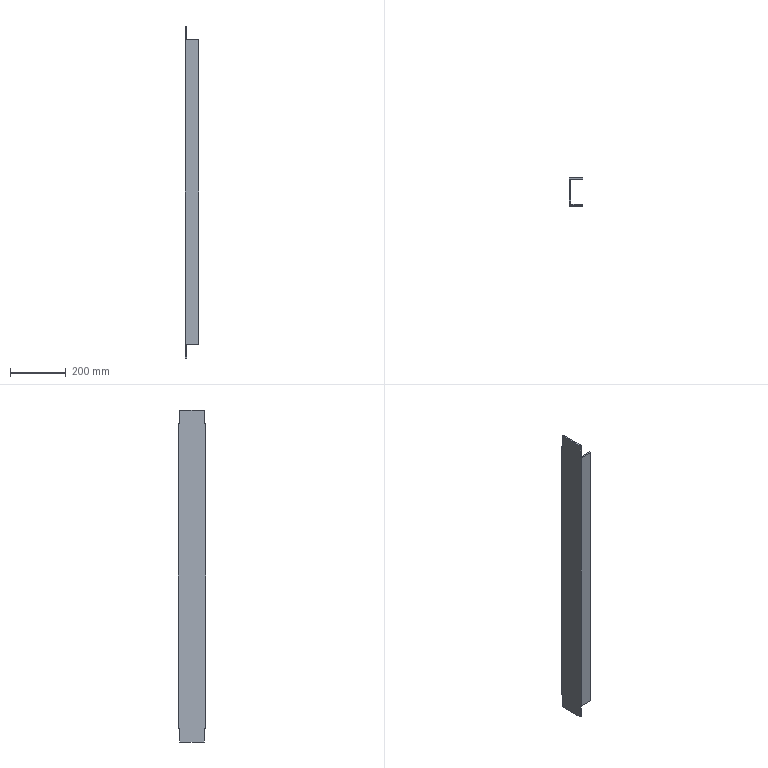Component | SolidWorks | 03LeftSideBase-2 | 1 solid | 28 faces | box 48 x 100 x 1189 mm | volume 1154848 mm3 | plane 18 | cylinder 10 | commonest cylinder face diameters 10 x10
build123d program:
from build123d import *

# Parameters (mm, degrees)
EXTRUDE_THIN1_DEPTH            = 1189
SKETCH2_W                      = 48
SKETCH2_H                      = 50
CUT_EXTRUDE1_DEPTH             = 5.5
SKETCH3_W                      = 48
SKETCH3_H                      = 50
CUT_EXTRUDE2_DEPTH             = 5.5
F_10_0_10_DIAMETER_HOLE1_D     = 10
F_10_0_10_DIAMETER_HOLE1_DEPTH = 5.5


with BuildPart() as part:
    # Sketch1 → Extrude-Thin1 (new body)
    with BuildSketch(Plane.XY):
        Polygon((48, 0), (0, 0), (0, 100), (48, 100), (48, 94.5), (5.5, 94.5), (5.5, 5.5), (48, 5.5), align=None)
    extrude(amount=EXTRUDE_THIN1_DEPTH)

    # Sketch2 → Cut-Extrude1 (cut)
    with BuildSketch(Plane(origin=(0, 100, 0), x_dir=(1, 0, 0), z_dir=(0, 1, 0))):
        with Locations((24, -1164)):
            Rectangle(SKETCH2_W, SKETCH2_H)
        with Locations((24, -25)):
            Rectangle(SKETCH2_W, SKETCH2_H)
    extrude(amount=-CUT_EXTRUDE1_DEPTH, mode=Mode.SUBTRACT)

    # Sketch3 → Cut-Extrude2 (cut)
    with BuildSketch(Plane.XZ):
        with Locations((24, 25)):
            Rectangle(SKETCH3_W, SKETCH3_H)
        with Locations((24, 1164)):
            Rectangle(SKETCH3_W, SKETCH3_H)
    extrude(amount=-CUT_EXTRUDE2_DEPTH, mode=Mode.SUBTRACT)

    # 10.0 _10_ Diameter Hole1
    with Locations(Plane(origin=(0, 100, 0), x_dir=(-1, 0, 0), z_dir=(0, 1, 0))):
        with Locations((-18, 194.5), (-18, 594.5), (-18, 994.5), (-18, 1126.5), (-18, 62.5)):
            Hole(F_10_0_10_DIAMETER_HOLE1_D / 2, depth=F_10_0_10_DIAMETER_HOLE1_DEPTH)


solid = part.part

# Placed as in the assembly
solid = solid.moved(Location((-123.527, -139.54, 42.607), (0, 0, 0)))
STEP:
#1=CARTESIAN_POINT('',(-4.155,-1.773,9.138));
#2=VERTEX_POINT('',#1);
#3=CARTESIAN_POINT('',(-4.155,-1.773,9.532));
#4=VERTEX_POINT('',#3);
#5=CARTESIAN_POINT('',(-4.155,-1.773,9.335));
#6=DIRECTION('',(0.,1.,0.));
#7=DIRECTION('',(0.,0.,1.));
#8=AXIS2_PLACEMENT_3D('',#5,#6,#7);
#9=CIRCLE('',#8,0.1969);
#10=EDGE_CURVE('',#2,#4,#9,.T.);
#11=ORIENTED_EDGE('',*,*,#10,.F.);
#12=CARTESIAN_POINT('',(-4.155,-1.557,9.138));
#13=VERTEX_POINT('',#12);
#14=CARTESIAN_POINT('',(-4.155,-1.557,9.138));
#15=DIRECTION('',(0.,1.,0.));
#16=VECTOR('',#15,39.37);
#17=LINE('',#14,#16);
#18=EDGE_CURVE('',#2,#13,#17,.T.);
#19=ORIENTED_EDGE('',*,*,#18,.T.);
#20=CARTESIAN_POINT('',(-4.155,-1.557,9.532));
#21=VERTEX_POINT('',#20);
#22=CARTESIAN_POINT('',(-4.155,-1.557,9.335));
#23=DIRECTION('',(0.,1.,0.));
#24=DIRECTION('',(0.,0.,1.));
#25=AXIS2_PLACEMENT_3D('',#22,#23,#24);
#26=CIRCLE('',#25,0.1969);
#27=EDGE_CURVE('',#13,#21,#26,.T.);
#28=ORIENTED_EDGE('',*,*,#27,.T.);
#29=CARTESIAN_POINT('',(-4.155,-1.557,9.532));
#30=DIRECTION('',(0.,1.,0.));
#31=VECTOR('',#30,39.37);
#32=LINE('',#29,#31);
#33=EDGE_CURVE('',#4,#21,#32,.T.);
#34=ORIENTED_EDGE('',*,*,#33,.F.);
#35=EDGE_LOOP('',(#11,#19,#28,#34));
#36=FACE_OUTER_BOUND('',#35,.T.);
#37=CARTESIAN_POINT('',(-4.155,-1.557,9.335));
#38=DIRECTION('',(0.,1.,0.));
#39=DIRECTION('',(0.,0.,1.));
#40=AXIS2_PLACEMENT_3D('',#37,#38,#39);
#41=CYLINDRICAL_SURFACE('',#40,0.1969);
#42=ADVANCED_FACE('',(#36),#41,.F.);
#43=CARTESIAN_POINT('',(-4.155,-1.773,24.886));
#44=VERTEX_POINT('',#43);
#45=CARTESIAN_POINT('',(-4.155,-1.773,25.28));
#46=VERTEX_POINT('',#45);
#47=CARTESIAN_POINT('',(-4.155,-1.773,25.083));
#48=DIRECTION('',(0.,1.,0.));
#49=DIRECTION('',(0.,0.,1.));
#50=AXIS2_PLACEMENT_3D('',#47,#48,#49);
#51=CIRCLE('',#50,0.1969);
#52=EDGE_CURVE('',#44,#46,#51,.T.);
#53=ORIENTED_EDGE('',*,*,#52,.F.);
#54=CARTESIAN_POINT('',(-4.155,-1.557,24.886));
#55=VERTEX_POINT('',#54);
#56=CARTESIAN_POINT('',(-4.155,-1.557,24.886));
#57=DIRECTION('',(0.,1.,0.));
#58=VECTOR('',#57,39.37);
#59=LINE('',#56,#58);
#60=EDGE_CURVE('',#44,#55,#59,.T.);
#61=ORIENTED_EDGE('',*,*,#60,.T.);
#62=CARTESIAN_POINT('',(-4.155,-1.557,25.28));
#63=VERTEX_POINT('',#62);
#64=CARTESIAN_POINT('',(-4.155,-1.557,25.083));
#65=DIRECTION('',(0.,1.,0.));
#66=DIRECTION('',(0.,0.,1.));
#67=AXIS2_PLACEMENT_3D('',#64,#65,#66);
#68=CIRCLE('',#67,0.1969);
#69=EDGE_CURVE('',#55,#63,#68,.T.);
#70=ORIENTED_EDGE('',*,*,#69,.T.);
#71=CARTESIAN_POINT('',(-4.155,-1.557,25.28));
#72=DIRECTION('',(0.,1.,0.));
#73=VECTOR('',#72,39.37);
#74=LINE('',#71,#73);
#75=EDGE_CURVE('',#46,#63,#74,.T.);
#76=ORIENTED_EDGE('',*,*,#75,.F.);
#77=EDGE_LOOP('',(#53,#61,#70,#76));
#78=FACE_OUTER_BOUND('',#77,.T.);
#79=CARTESIAN_POINT('',(-4.155,-1.557,25.083));
#80=DIRECTION('',(0.,1.,0.));
#81=DIRECTION('',(0.,0.,1.));
#82=AXIS2_PLACEMENT_3D('',#79,#80,#81);
#83=CYLINDRICAL_SURFACE('',#82,0.1969);
#84=ADVANCED_FACE('',(#78),#83,.F.);
#85=CARTESIAN_POINT('',(-4.155,-1.773,40.634));
#86=VERTEX_POINT('',#85);
#87=CARTESIAN_POINT('',(-4.155,-1.773,41.028));
#88=VERTEX_POINT('',#87);
#89=CARTESIAN_POINT('',(-4.155,-1.773,40.831));
#90=DIRECTION('',(0.,1.,0.));
#91=DIRECTION('',(0.,0.,1.));
#92=AXIS2_PLACEMENT_3D('',#89,#90,#91);
#93=CIRCLE('',#92,0.1969);
#94=EDGE_CURVE('',#86,#88,#93,.T.);
#95=ORIENTED_EDGE('',*,*,#94,.F.);
#96=CARTESIAN_POINT('',(-4.155,-1.557,40.634));
#97=VERTEX_POINT('',#96);
#98=CARTESIAN_POINT('',(-4.155,-1.557,40.634));
#99=DIRECTION('',(0.,1.,0.));
#100=VECTOR('',#99,39.37);
#101=LINE('',#98,#100);
#102=EDGE_CURVE('',#86,#97,#101,.T.);
#103=ORIENTED_EDGE('',*,*,#102,.T.);
#104=CARTESIAN_POINT('',(-4.155,-1.557,41.028));
#105=VERTEX_POINT('',#104);
#106=CARTESIAN_POINT('',(-4.155,-1.557,40.831));
#107=DIRECTION('',(0.,1.,0.));
#108=DIRECTION('',(0.,0.,1.));
#109=AXIS2_PLACEMENT_3D('',#106,#107,#108);
#110=CIRCLE('',#109,0.1969);
#111=EDGE_CURVE('',#97,#105,#110,.T.);
#112=ORIENTED_EDGE('',*,*,#111,.T.);
#113=CARTESIAN_POINT('',(-4.155,-1.557,41.028));
#114=DIRECTION('',(0.,1.,0.));
#115=VECTOR('',#114,39.37);
#116=LINE('',#113,#115);
#117=EDGE_CURVE('',#88,#105,#116,.T.);
#118=ORIENTED_EDGE('',*,*,#117,.F.);
#119=EDGE_LOOP('',(#95,#103,#112,#118));
#120=FACE_OUTER_BOUND('',#119,.T.);
#121=CARTESIAN_POINT('',(-4.155,-1.557,40.831));
#122=DIRECTION('',(0.,1.,0.));
#123=DIRECTION('',(0.,0.,1.));
#124=AXIS2_PLACEMENT_3D('',#121,#122,#123);
#125=CYLINDRICAL_SURFACE('',#124,0.1969);
#126=ADVANCED_FACE('',(#120),#125,.F.);
#127=CARTESIAN_POINT('',(-4.155,-1.773,45.831));
#128=VERTEX_POINT('',#127);
#129=CARTESIAN_POINT('',(-4.155,-1.773,46.225));
#130=VERTEX_POINT('',#129);
#131=CARTESIAN_POINT('',(-4.155,-1.773,46.028));
#132=DIRECTION('',(0.,1.,0.));
#133=DIRECTION('',(0.,0.,1.));
#134=AXIS2_PLACEMENT_3D('',#131,#132,#133);
#135=CIRCLE('',#134,0.1969);
#136=EDGE_CURVE('',#128,#130,#135,.T.);
#137=ORIENTED_EDGE('',*,*,#136,.F.);
#138=CARTESIAN_POINT('',(-4.155,-1.557,45.831));
#139=VERTEX_POINT('',#138);
#140=CARTESIAN_POINT('',(-4.155,-1.557,45.831));
#141=DIRECTION('',(0.,1.,0.));
#142=VECTOR('',#141,39.37);
#143=LINE('',#140,#142);
#144=EDGE_CURVE('',#128,#139,#143,.T.);
#145=ORIENTED_EDGE('',*,*,#144,.T.);
#146=CARTESIAN_POINT('',(-4.155,-1.557,46.225));
#147=VERTEX_POINT('',#146);
#148=CARTESIAN_POINT('',(-4.155,-1.557,46.028));
#149=DIRECTION('',(0.,1.,0.));
#150=DIRECTION('',(0.,0.,1.));
#151=AXIS2_PLACEMENT_3D('',#148,#149,#150);
#152=CIRCLE('',#151,0.1969);
#153=EDGE_CURVE('',#139,#147,#152,.T.);
#154=ORIENTED_EDGE('',*,*,#153,.T.);
#155=CARTESIAN_POINT('',(-4.155,-1.557,46.225));
#156=DIRECTION('',(0.,1.,0.));
#157=VECTOR('',#156,39.37);
#158=LINE('',#155,#157);
#159=EDGE_CURVE('',#130,#147,#158,.T.);
#160=ORIENTED_EDGE('',*,*,#159,.F.);
#161=EDGE_LOOP('',(#137,#145,#154,#160));
#162=FACE_OUTER_BOUND('',#161,.T.);
#163=CARTESIAN_POINT('',(-4.155,-1.557,46.028));
#164=DIRECTION('',(0.,1.,0.));
#165=DIRECTION('',(0.,0.,1.));
#166=AXIS2_PLACEMENT_3D('',#163,#164,#165);
#167=CYLINDRICAL_SURFACE('',#166,0.1969);
#168=ADVANCED_FACE('',(#162),#167,.F.);
#169=CARTESIAN_POINT('',(-4.155,-1.773,3.941));
#170=VERTEX_POINT('',#169);
#171=CARTESIAN_POINT('',(-4.155,-1.773,4.335));
#172=VERTEX_POINT('',#171);
#173=CARTESIAN_POINT('',(-4.155,-1.773,4.138));
#174=DIRECTION('',(0.,1.,0.));
#175=DIRECTION('',(0.,0.,1.));
#176=AXIS2_PLACEMENT_3D('',#173,#174,#175);
#177=CIRCLE('',#176,0.1969);
#178=EDGE_CURVE('',#170,#172,#177,.T.);
#179=ORIENTED_EDGE('',*,*,#178,.F.);
#180=CARTESIAN_POINT('',(-4.155,-1.557,3.941));
#181=VERTEX_POINT('',#180);
#182=CARTESIAN_POINT('',(-4.155,-1.557,3.941));
#183=DIRECTION('',(0.,1.,0.));
#184=VECTOR('',#183,39.37);
#185=LINE('',#182,#184);
#186=EDGE_CURVE('',#170,#181,#185,.T.);
#187=ORIENTED_EDGE('',*,*,#186,.T.);
#188=CARTESIAN_POINT('',(-4.155,-1.557,4.335));
#189=VERTEX_POINT('',#188);
#190=CARTESIAN_POINT('',(-4.155,-1.557,4.138));
#191=DIRECTION('',(0.,1.,0.));
#192=DIRECTION('',(0.,0.,1.));
#193=AXIS2_PLACEMENT_3D('',#190,#191,#192);
#194=CIRCLE('',#193,0.1969);
#195=EDGE_CURVE('',#181,#189,#194,.T.);
#196=ORIENTED_EDGE('',*,*,#195,.T.);
#197=CARTESIAN_POINT('',(-4.155,-1.557,4.335));
#198=DIRECTION('',(0.,1.,0.));
#199=VECTOR('',#198,39.37);
#200=LINE('',#197,#199);
#201=EDGE_CURVE('',#172,#189,#200,.T.);
#202=ORIENTED_EDGE('',*,*,#201,.F.);
#203=EDGE_LOOP('',(#179,#187,#196,#202));
#204=FACE_OUTER_BOUND('',#203,.T.);
#205=CARTESIAN_POINT('',(-4.155,-1.557,4.138));
#206=DIRECTION('',(0.,1.,0.));
#207=DIRECTION('',(0.,0.,1.));
#208=AXIS2_PLACEMENT_3D('',#205,#206,#207);
#209=CYLINDRICAL_SURFACE('',#208,0.1969);
#210=ADVANCED_FACE('',(#204),#209,.F.);
#211=CARTESIAN_POINT('',(-4.863,-5.277,48.488));
#212=VERTEX_POINT('',#211);
#213=CARTESIAN_POINT('',(-4.647,-5.277,48.488));
#214=VERTEX_POINT('',#213);
#215=CARTESIAN_POINT('',(-2.974,-5.277,48.488));
#216=DIRECTION('',(1.,-0.,0.));
#217=VECTOR('',#216,39.37);
#218=LINE('',#215,#217);
#219=EDGE_CURVE('',#212,#214,#218,.T.);
#220=ORIENTED_EDGE('',*,*,#219,.T.);
#221=CARTESIAN_POINT('',(-4.647,-1.773,48.488));
#222=VERTEX_POINT('',#221);
#223=CARTESIAN_POINT('',(-4.647,-5.494,48.488));
#224=DIRECTION('',(0.,1.,0.));
#225=VECTOR('',#224,39.37);
#226=LINE('',#223,#225);
#227=EDGE_CURVE('',#214,#222,#226,.T.);
#228=ORIENTED_EDGE('',*,*,#227,.T.);
#229=CARTESIAN_POINT('',(-4.863,-1.773,48.488));
#230=VERTEX_POINT('',#229);
#231=CARTESIAN_POINT('',(-2.974,-1.773,48.488));
#232=DIRECTION('',(1.,0.,0.));
#233=VECTOR('',#232,39.37);
#234=LINE('',#231,#233);
#235=EDGE_CURVE('',#230,#222,#234,.T.);
#236=ORIENTED_EDGE('',*,*,#235,.F.);
#237=CARTESIAN_POINT('',(-4.863,-5.494,48.488));
#238=DIRECTION('',(0.,1.,0.));
#239=VECTOR('',#238,39.37);
#240=LINE('',#237,#239);
#241=EDGE_CURVE('',#212,#230,#240,.T.);
#242=ORIENTED_EDGE('',*,*,#241,.F.);
#243=EDGE_LOOP('',(#220,#228,#236,#242));
#244=FACE_OUTER_BOUND('',#243,.T.);
#245=CARTESIAN_POINT('',(-2.974,-1.773,48.488));
#246=DIRECTION('',(0.,0.,-1.));
#247=DIRECTION('',(-1.,0.,0.));
#248=AXIS2_PLACEMENT_3D('',#245,#246,#247);
#249=PLANE('',#248);
#250=ADVANCED_FACE('',(#244),#249,.F.);
#251=CARTESIAN_POINT('',(-4.647,-5.277,1.677));
#252=VERTEX_POINT('',#251);
#253=CARTESIAN_POINT('',(-4.647,-1.773,1.677));
#254=VERTEX_POINT('',#253);
#255=CARTESIAN_POINT('',(-4.647,-5.494,1.677));
#256=DIRECTION('',(0.,1.,0.));
#257=VECTOR('',#256,39.37);
#258=LINE('',#255,#257);
#259=EDGE_CURVE('',#252,#254,#258,.T.);
#260=ORIENTED_EDGE('',*,*,#259,.F.);
#261=CARTESIAN_POINT('',(-4.863,-5.277,1.677));
#262=VERTEX_POINT('',#261);
#263=CARTESIAN_POINT('',(-2.974,-5.277,1.677));
#264=DIRECTION('',(-1.,0.,0.));
#265=VECTOR('',#264,39.37);
#266=LINE('',#263,#265);
#267=EDGE_CURVE('',#252,#262,#266,.T.);
#268=ORIENTED_EDGE('',*,*,#267,.T.);
#269=CARTESIAN_POINT('',(-4.863,-1.773,1.677));
#270=VERTEX_POINT('',#269);
#271=CARTESIAN_POINT('',(-4.863,-5.494,1.677));
#272=DIRECTION('',(0.,1.,0.));
#273=VECTOR('',#272,39.37);
#274=LINE('',#271,#273);
#275=EDGE_CURVE('',#262,#270,#274,.T.);
#276=ORIENTED_EDGE('',*,*,#275,.T.);
#277=CARTESIAN_POINT('',(-2.974,-1.773,1.677));
#278=DIRECTION('',(1.,0.,0.));
#279=VECTOR('',#278,39.37);
#280=LINE('',#277,#279);
#281=EDGE_CURVE('',#270,#254,#280,.T.);
#282=ORIENTED_EDGE('',*,*,#281,.T.);
#283=EDGE_LOOP('',(#260,#268,#276,#282));
#284=FACE_OUTER_BOUND('',#283,.T.);
#285=CARTESIAN_POINT('',(-2.974,-1.773,1.677));
#286=DIRECTION('',(0.,0.,-1.));
#287=DIRECTION('',(-1.,0.,0.));
#288=AXIS2_PLACEMENT_3D('',#285,#286,#287);
#289=PLANE('',#288);
#290=ADVANCED_FACE('',(#284),#289,.T.);
#291=CARTESIAN_POINT('',(-4.155,-1.773,9.335));
#292=DIRECTION('',(0.,1.,0.));
#293=DIRECTION('',(0.,0.,1.));
#294=AXIS2_PLACEMENT_3D('',#291,#292,#293);
#295=CIRCLE('',#294,0.1969);
#296=EDGE_CURVE('',#4,#2,#295,.T.);
#297=ORIENTED_EDGE('',*,*,#296,.T.);
#298=ORIENTED_EDGE('',*,*,#10,.T.);
#299=EDGE_LOOP('',(#297,#298));
#300=FACE_BOUND('',#299,.T.);
#301=CARTESIAN_POINT('',(-4.155,-1.773,25.083));
#302=DIRECTION('',(0.,1.,0.));
#303=DIRECTION('',(0.,0.,1.));
#304=AXIS2_PLACEMENT_3D('',#301,#302,#303);
#305=CIRCLE('',#304,0.1969);
#306=EDGE_CURVE('',#46,#44,#305,.T.);
#307=ORIENTED_EDGE('',*,*,#306,.T.);
#308=ORIENTED_EDGE('',*,*,#52,.T.);
#309=EDGE_LOOP('',(#307,#308));
#310=FACE_BOUND('',#309,.T.);
#311=CARTESIAN_POINT('',(-4.155,-1.773,40.831));
#312=DIRECTION('',(0.,1.,0.));
#313=DIRECTION('',(0.,0.,1.));
#314=AXIS2_PLACEMENT_3D('',#311,#312,#313);
#315=CIRCLE('',#314,0.1969);
#316=EDGE_CURVE('',#88,#86,#315,.T.);
#317=ORIENTED_EDGE('',*,*,#316,.T.);
#318=ORIENTED_EDGE('',*,*,#94,.T.);
#319=EDGE_LOOP('',(#317,#318));
#320=FACE_BOUND('',#319,.T.);
#321=CARTESIAN_POINT('',(-4.155,-1.773,46.028));
#322=DIRECTION('',(0.,1.,0.));
#323=DIRECTION('',(0.,0.,1.));
#324=AXIS2_PLACEMENT_3D('',#321,#322,#323);
#325=CIRCLE('',#324,0.1969);
#326=EDGE_CURVE('',#130,#128,#325,.T.);
#327=ORIENTED_EDGE('',*,*,#326,.T.);
#328=ORIENTED_EDGE('',*,*,#136,.T.);
#329=EDGE_LOOP('',(#327,#328));
#330=FACE_BOUND('',#329,.T.);
#331=CARTESIAN_POINT('',(-4.155,-1.773,4.138));
#332=DIRECTION('',(0.,1.,0.));
#333=DIRECTION('',(0.,0.,1.));
#334=AXIS2_PLACEMENT_3D('',#331,#332,#333);
#335=CIRCLE('',#334,0.1969);
#336=EDGE_CURVE('',#172,#170,#335,.T.);
#337=ORIENTED_EDGE('',*,*,#336,.T.);
#338=ORIENTED_EDGE('',*,*,#178,.T.);
#339=EDGE_LOOP('',(#337,#338));
#340=FACE_BOUND('',#339,.T.);
#341=CARTESIAN_POINT('',(-4.647,-1.773,46.52));
#342=VERTEX_POINT('',#341);
#343=CARTESIAN_POINT('',(-4.647,-1.773,3.646));
#344=VERTEX_POINT('',#343);
#345=CARTESIAN_POINT('',(-4.647,-1.773,48.488));
#346=DIRECTION('',(0.,0.,-1.));
#347=VECTOR('',#346,39.37);
#348=LINE('',#345,#347);
#349=EDGE_CURVE('',#342,#344,#348,.T.);
#350=ORIENTED_EDGE('',*,*,#349,.T.);
#351=CARTESIAN_POINT('',(-2.974,-1.773,3.646));
#352=VERTEX_POINT('',#351);
#353=CARTESIAN_POINT('',(-2.974,-1.773,3.646));
#354=DIRECTION('',(-1.,0.,0.));
#355=VECTOR('',#354,39.37);
#356=LINE('',#353,#355);
#357=EDGE_CURVE('',#352,#344,#356,.T.);
#358=ORIENTED_EDGE('',*,*,#357,.F.);
#359=CARTESIAN_POINT('',(-2.974,-1.773,46.52));
#360=VERTEX_POINT('',#359);
#361=CARTESIAN_POINT('',(-2.974,-1.773,48.488));
#362=DIRECTION('',(0.,0.,-1.));
#363=VECTOR('',#362,39.37);
#364=LINE('',#361,#363);
#365=EDGE_CURVE('',#360,#352,#364,.T.);
#366=ORIENTED_EDGE('',*,*,#365,.F.);
#367=CARTESIAN_POINT('',(-2.974,-1.773,46.52));
#368=DIRECTION('',(1.,0.,0.));
#369=VECTOR('',#368,39.37);
#370=LINE('',#367,#369);
#371=EDGE_CURVE('',#342,#360,#370,.T.);
#372=ORIENTED_EDGE('',*,*,#371,.F.);
#373=EDGE_LOOP('',(#350,#358,#366,#372));
#374=FACE_OUTER_BOUND('',#373,.T.);
#375=CARTESIAN_POINT('',(-4.863,-1.773,48.488));
#376=DIRECTION('',(0.,1.,0.));
#377=DIRECTION('',(0.,0.,1.));
#378=AXIS2_PLACEMENT_3D('',#375,#376,#377);
#379=PLANE('',#378);
#380=ADVANCED_FACE('',(#300,#310,#320,#330,#340,#374),#379,.F.);
#381=CARTESIAN_POINT('',(-2.974,-1.557,3.646));
#382=VERTEX_POINT('',#381);
#383=CARTESIAN_POINT('',(-2.974,-4.502,3.646));
#384=DIRECTION('',(0.,1.,0.));
#385=VECTOR('',#384,39.37);
#386=LINE('',#383,#385);
#387=EDGE_CURVE('',#352,#382,#386,.T.);
#388=ORIENTED_EDGE('',*,*,#387,.T.);
#389=CARTESIAN_POINT('',(-2.974,-1.557,46.52));
#390=VERTEX_POINT('',#389);
#391=CARTESIAN_POINT('',(-2.974,-1.557,48.488));
#392=DIRECTION('',(0.,0.,-1.));
#393=VECTOR('',#392,39.37);
#394=LINE('',#391,#393);
#395=EDGE_CURVE('',#390,#382,#394,.T.);
#396=ORIENTED_EDGE('',*,*,#395,.F.);
#397=CARTESIAN_POINT('',(-2.974,-4.502,46.52));
#398=DIRECTION('',(0.,1.,0.));
#399=VECTOR('',#398,39.37);
#400=LINE('',#397,#399);
#401=EDGE_CURVE('',#360,#390,#400,.T.);
#402=ORIENTED_EDGE('',*,*,#401,.F.);
#403=ORIENTED_EDGE('',*,*,#365,.T.);
#404=EDGE_LOOP('',(#388,#396,#402,#403));
#405=FACE_OUTER_BOUND('',#404,.T.);
#406=CARTESIAN_POINT('',(-2.974,-1.557,48.488));
#407=DIRECTION('',(1.,0.,0.));
#408=DIRECTION('',(0.,0.,-1.));
#409=AXIS2_PLACEMENT_3D('',#406,#407,#408);
#410=PLANE('',#409);
#411=ADVANCED_FACE('',(#405),#410,.T.);
#412=CARTESIAN_POINT('',(-4.155,-1.557,9.335));
#413=DIRECTION('',(0.,1.,0.));
#414=DIRECTION('',(0.,0.,1.));
#415=AXIS2_PLACEMENT_3D('',#412,#413,#414);
#416=CIRCLE('',#415,0.1969);
#417=EDGE_CURVE('',#21,#13,#416,.T.);
#418=ORIENTED_EDGE('',*,*,#417,.F.);
#419=ORIENTED_EDGE('',*,*,#27,.F.);
#420=EDGE_LOOP('',(#418,#419));
#421=FACE_BOUND('',#420,.T.);
#422=CARTESIAN_POINT('',(-4.155,-1.557,25.083));
#423=DIRECTION('',(0.,1.,0.));
#424=DIRECTION('',(0.,0.,1.));
#425=AXIS2_PLACEMENT_3D('',#422,#423,#424);
#426=CIRCLE('',#425,0.1969);
#427=EDGE_CURVE('',#63,#55,#426,.T.);
#428=ORIENTED_EDGE('',*,*,#427,.F.);
#429=ORIENTED_EDGE('',*,*,#69,.F.);
#430=EDGE_LOOP('',(#428,#429));
#431=FACE_BOUND('',#430,.T.);
#432=CARTESIAN_POINT('',(-4.155,-1.557,40.831));
#433=DIRECTION('',(0.,1.,0.));
#434=DIRECTION('',(0.,0.,1.));
#435=AXIS2_PLACEMENT_3D('',#432,#433,#434);
#436=CIRCLE('',#435,0.1969);
#437=EDGE_CURVE('',#105,#97,#436,.T.);
#438=ORIENTED_EDGE('',*,*,#437,.F.);
#439=ORIENTED_EDGE('',*,*,#111,.F.);
#440=EDGE_LOOP('',(#438,#439));
#441=FACE_BOUND('',#440,.T.);
#442=CARTESIAN_POINT('',(-4.155,-1.557,46.028));
#443=DIRECTION('',(0.,1.,0.));
#444=DIRECTION('',(0.,0.,1.));
#445=AXIS2_PLACEMENT_3D('',#442,#443,#444);
#446=CIRCLE('',#445,0.1969);
#447=EDGE_CURVE('',#147,#139,#446,.T.);
#448=ORIENTED_EDGE('',*,*,#447,.F.);
#449=ORIENTED_EDGE('',*,*,#153,.F.);
#450=EDGE_LOOP('',(#448,#449));
#451=FACE_BOUND('',#450,.T.);
#452=CARTESIAN_POINT('',(-4.155,-1.557,4.138));
#453=DIRECTION('',(0.,1.,0.));
#454=DIRECTION('',(0.,0.,1.));
#455=AXIS2_PLACEMENT_3D('',#452,#453,#454);
#456=CIRCLE('',#455,0.1969);
#457=EDGE_CURVE('',#189,#181,#456,.T.);
#458=ORIENTED_EDGE('',*,*,#457,.F.);
#459=ORIENTED_EDGE('',*,*,#195,.F.);
#460=EDGE_LOOP('',(#458,#459));
#461=FACE_BOUND('',#460,.T.);
#462=CARTESIAN_POINT('',(-4.863,-1.557,3.646));
#463=VERTEX_POINT('',#462);
#464=CARTESIAN_POINT('',(-2.974,-1.557,3.646));
#465=DIRECTION('',(1.,0.,0.));
#466=VECTOR('',#465,39.37);
#467=LINE('',#464,#466);
#468=EDGE_CURVE('',#463,#382,#467,.T.);
#469=ORIENTED_EDGE('',*,*,#468,.F.);
#470=CARTESIAN_POINT('',(-4.863,-1.557,46.52));
#471=VERTEX_POINT('',#470);
#472=CARTESIAN_POINT('',(-4.863,-1.557,48.488));
#473=DIRECTION('',(0.,0.,-1.));
#474=VECTOR('',#473,39.37);
#475=LINE('',#472,#474);
#476=EDGE_CURVE('',#471,#463,#475,.T.);
#477=ORIENTED_EDGE('',*,*,#476,.F.);
#478=CARTESIAN_POINT('',(-2.974,-1.557,46.52));
#479=DIRECTION('',(-1.,0.,0.));
#480=VECTOR('',#479,39.37);
#481=LINE('',#478,#480);
#482=EDGE_CURVE('',#390,#471,#481,.T.);
#483=ORIENTED_EDGE('',*,*,#482,.F.);
#484=ORIENTED_EDGE('',*,*,#395,.T.);
#485=EDGE_LOOP('',(#469,#477,#483,#484));
#486=FACE_OUTER_BOUND('',#485,.T.);
#487=CARTESIAN_POINT('',(-4.863,-1.557,48.488));
#488=DIRECTION('',(0.,1.,0.));
#489=DIRECTION('',(0.,0.,1.));
#490=AXIS2_PLACEMENT_3D('',#487,#488,#489);
#491=PLANE('',#490);
#492=ADVANCED_FACE('',(#421,#431,#441,#451,#461,#486),#491,.T.);
#493=CARTESIAN_POINT('',(-4.863,-5.277,46.52));
#494=VERTEX_POINT('',#493);
#495=CARTESIAN_POINT('',(-4.863,-5.494,46.52));
#496=VERTEX_POINT('',#495);
#497=CARTESIAN_POINT('',(-4.863,-2.548,46.52));
#498=DIRECTION('',(-0.,-1.,0.));
#499=VECTOR('',#498,39.37);
#500=LINE('',#497,#499);
#501=EDGE_CURVE('',#494,#496,#500,.T.);
#502=ORIENTED_EDGE('',*,*,#501,.F.);
#503=CARTESIAN_POINT('',(-4.863,-5.277,48.488));
#504=DIRECTION('',(0.,0.,1.));
#505=VECTOR('',#504,39.37);
#506=LINE('',#503,#505);
#507=EDGE_CURVE('',#494,#212,#506,.T.);
#508=ORIENTED_EDGE('',*,*,#507,.T.);
#509=ORIENTED_EDGE('',*,*,#241,.T.);
#510=CARTESIAN_POINT('',(-4.863,-1.773,46.52));
#511=VERTEX_POINT('',#510);
#512=CARTESIAN_POINT('',(-4.863,-1.773,48.488));
#513=DIRECTION('',(0.,0.,-1.));
#514=VECTOR('',#513,39.37);
#515=LINE('',#512,#514);
#516=EDGE_CURVE('',#230,#511,#515,.T.);
#517=ORIENTED_EDGE('',*,*,#516,.T.);
#518=CARTESIAN_POINT('',(-4.863,-4.502,46.52));
#519=DIRECTION('',(0.,1.,0.));
#520=VECTOR('',#519,39.37);
#521=LINE('',#518,#520);
#522=EDGE_CURVE('',#511,#471,#521,.T.);
#523=ORIENTED_EDGE('',*,*,#522,.T.);
#524=ORIENTED_EDGE('',*,*,#476,.T.);
#525=CARTESIAN_POINT('',(-4.863,-1.773,3.646));
#526=VERTEX_POINT('',#525);
#527=CARTESIAN_POINT('',(-4.863,-4.502,3.646));
#528=DIRECTION('',(0.,1.,0.));
#529=VECTOR('',#528,39.37);
#530=LINE('',#527,#529);
#531=EDGE_CURVE('',#526,#463,#530,.T.);
#532=ORIENTED_EDGE('',*,*,#531,.F.);
#533=CARTESIAN_POINT('',(-4.863,-1.773,1.677));
#534=DIRECTION('',(0.,0.,-1.));
#535=VECTOR('',#534,39.37);
#536=LINE('',#533,#535);
#537=EDGE_CURVE('',#526,#270,#536,.T.);
#538=ORIENTED_EDGE('',*,*,#537,.T.);
#539=ORIENTED_EDGE('',*,*,#275,.F.);
#540=CARTESIAN_POINT('',(-4.863,-5.277,3.646));
#541=VERTEX_POINT('',#540);
#542=CARTESIAN_POINT('',(-4.863,-5.277,1.677));
#543=DIRECTION('',(0.,0.,1.));
#544=VECTOR('',#543,39.37);
#545=LINE('',#542,#544);
#546=EDGE_CURVE('',#262,#541,#545,.T.);
#547=ORIENTED_EDGE('',*,*,#546,.T.);
#548=CARTESIAN_POINT('',(-4.863,-5.494,3.646));
#549=VERTEX_POINT('',#548);
#550=CARTESIAN_POINT('',(-4.863,-2.548,3.646));
#551=DIRECTION('',(-0.,-1.,0.));
#552=VECTOR('',#551,39.37);
#553=LINE('',#550,#552);
#554=EDGE_CURVE('',#541,#549,#553,.T.);
#555=ORIENTED_EDGE('',*,*,#554,.T.);
#556=CARTESIAN_POINT('',(-4.863,-5.494,48.488));
#557=DIRECTION('',(0.,0.,-1.));
#558=VECTOR('',#557,39.37);
#559=LINE('',#556,#558);
#560=EDGE_CURVE('',#496,#549,#559,.T.);
#561=ORIENTED_EDGE('',*,*,#560,.F.);
#562=EDGE_LOOP('',(#502,#508,#509,#517,#523,#524,#532,#538,#539,#547,#555,#561));
#563=FACE_OUTER_BOUND('',#562,.T.);
#564=CARTESIAN_POINT('',(-4.863,-5.494,48.488));
#565=DIRECTION('',(-1.,0.,0.));
#566=DIRECTION('',(0.,0.,1.));
#567=AXIS2_PLACEMENT_3D('',#564,#565,#566);
#568=PLANE('',#567);
#569=ADVANCED_FACE('',(#563),#568,.T.);
#570=CARTESIAN_POINT('',(-2.974,-5.494,46.52));
#571=VERTEX_POINT('',#570);
#572=CARTESIAN_POINT('',(-2.974,-5.494,46.52));
#573=DIRECTION('',(1.,-0.,0.));
#574=VECTOR('',#573,39.37);
#575=LINE('',#572,#574);
#576=EDGE_CURVE('',#496,#571,#575,.T.);
#577=ORIENTED_EDGE('',*,*,#576,.F.);
#578=ORIENTED_EDGE('',*,*,#560,.T.);
#579=CARTESIAN_POINT('',(-2.974,-5.494,3.646));
#580=VERTEX_POINT('',#579);
#581=CARTESIAN_POINT('',(-2.974,-5.494,3.646));
#582=DIRECTION('',(-1.,0.,0.));
#583=VECTOR('',#582,39.37);
#584=LINE('',#581,#583);
#585=EDGE_CURVE('',#580,#549,#584,.T.);
#586=ORIENTED_EDGE('',*,*,#585,.F.);
#587=CARTESIAN_POINT('',(-2.974,-5.494,48.488));
#588=DIRECTION('',(0.,0.,-1.));
#589=VECTOR('',#588,39.37);
#590=LINE('',#587,#589);
#591=EDGE_CURVE('',#571,#580,#590,.T.);
#592=ORIENTED_EDGE('',*,*,#591,.F.);
#593=EDGE_LOOP('',(#577,#578,#586,#592));
#594=FACE_OUTER_BOUND('',#593,.T.);
#595=CARTESIAN_POINT('',(-2.974,-5.494,48.488));
#596=DIRECTION('',(-0.,-1.,0.));
#597=DIRECTION('',(1.,-0.,0.));
#598=AXIS2_PLACEMENT_3D('',#595,#596,#597);
#599=PLANE('',#598);
#600=ADVANCED_FACE('',(#594),#599,.T.);
#601=CARTESIAN_POINT('',(-2.974,-5.277,46.52));
#602=VERTEX_POINT('',#601);
#603=CARTESIAN_POINT('',(-2.974,-2.548,46.52));
#604=DIRECTION('',(-0.,-1.,0.));
#605=VECTOR('',#604,39.37);
#606=LINE('',#603,#605);
#607=EDGE_CURVE('',#602,#571,#606,.T.);
#608=ORIENTED_EDGE('',*,*,#607,.T.);
#609=ORIENTED_EDGE('',*,*,#591,.T.);
#610=CARTESIAN_POINT('',(-2.974,-5.277,3.646));
#611=VERTEX_POINT('',#610);
#612=CARTESIAN_POINT('',(-2.974,-2.548,3.646));
#613=DIRECTION('',(-0.,-1.,0.));
#614=VECTOR('',#613,39.37);
#615=LINE('',#612,#614);
#616=EDGE_CURVE('',#611,#580,#615,.T.);
#617=ORIENTED_EDGE('',*,*,#616,.F.);
#618=CARTESIAN_POINT('',(-2.974,-5.277,48.488));
#619=DIRECTION('',(0.,0.,-1.));
#620=VECTOR('',#619,39.37);
#621=LINE('',#618,#620);
#622=EDGE_CURVE('',#602,#611,#621,.T.);
#623=ORIENTED_EDGE('',*,*,#622,.F.);
#624=EDGE_LOOP('',(#608,#609,#617,#623));
#625=FACE_OUTER_BOUND('',#624,.T.);
#626=CARTESIAN_POINT('',(-2.974,-5.277,48.488));
#627=DIRECTION('',(1.,0.,0.));
#628=DIRECTION('',(0.,0.,-1.));
#629=AXIS2_PLACEMENT_3D('',#626,#627,#628);
#630=PLANE('',#629);
#631=ADVANCED_FACE('',(#625),#630,.T.);
#632=CARTESIAN_POINT('',(-4.647,-5.277,46.52));
#633=VERTEX_POINT('',#632);
#634=CARTESIAN_POINT('',(-4.647,-5.277,3.646));
#635=VERTEX_POINT('',#634);
#636=CARTESIAN_POINT('',(-4.647,-5.277,48.488));
#637=DIRECTION('',(0.,0.,-1.));
#638=VECTOR('',#637,39.37);
#639=LINE('',#636,#638);
#640=EDGE_CURVE('',#633,#635,#639,.T.);
#641=ORIENTED_EDGE('',*,*,#640,.F.);
#642=CARTESIAN_POINT('',(-2.974,-5.277,46.52));
#643=DIRECTION('',(-1.,0.,0.));
#644=VECTOR('',#643,39.37);
#645=LINE('',#642,#644);
#646=EDGE_CURVE('',#602,#633,#645,.T.);
#647=ORIENTED_EDGE('',*,*,#646,.F.);
#648=ORIENTED_EDGE('',*,*,#622,.T.);
#649=CARTESIAN_POINT('',(-2.974,-5.277,3.646));
#650=DIRECTION('',(1.,-0.,0.));
#651=VECTOR('',#650,39.37);
#652=LINE('',#649,#651);
#653=EDGE_CURVE('',#635,#611,#652,.T.);
#654=ORIENTED_EDGE('',*,*,#653,.F.);
#655=EDGE_LOOP('',(#641,#647,#648,#654));
#656=FACE_OUTER_BOUND('',#655,.T.);
#657=CARTESIAN_POINT('',(-2.974,-5.277,48.488));
#658=DIRECTION('',(-0.,-1.,0.));
#659=DIRECTION('',(1.,-0.,0.));
#660=AXIS2_PLACEMENT_3D('',#657,#658,#659);
#661=PLANE('',#660);
#662=ADVANCED_FACE('',(#656),#661,.F.);
#663=ORIENTED_EDGE('',*,*,#259,.T.);
#664=CARTESIAN_POINT('',(-4.647,-1.773,48.488));
#665=DIRECTION('',(0.,0.,-1.));
#666=VECTOR('',#665,39.37);
#667=LINE('',#664,#666);
#668=EDGE_CURVE('',#344,#254,#667,.T.);
#669=ORIENTED_EDGE('',*,*,#668,.F.);
#670=ORIENTED_EDGE('',*,*,#349,.F.);
#671=CARTESIAN_POINT('',(-4.647,-1.773,48.488));
#672=DIRECTION('',(0.,0.,-1.));
#673=VECTOR('',#672,39.37);
#674=LINE('',#671,#673);
#675=EDGE_CURVE('',#222,#342,#674,.T.);
#676=ORIENTED_EDGE('',*,*,#675,.F.);
#677=ORIENTED_EDGE('',*,*,#227,.F.);
#678=CARTESIAN_POINT('',(-4.647,-5.277,48.488));
#679=DIRECTION('',(0.,0.,-1.));
#680=VECTOR('',#679,39.37);
#681=LINE('',#678,#680);
#682=EDGE_CURVE('',#214,#633,#681,.T.);
#683=ORIENTED_EDGE('',*,*,#682,.T.);
#684=ORIENTED_EDGE('',*,*,#640,.T.);
#685=CARTESIAN_POINT('',(-4.647,-5.277,48.488));
#686=DIRECTION('',(0.,0.,-1.));
#687=VECTOR('',#686,39.37);
#688=LINE('',#685,#687);
#689=EDGE_CURVE('',#635,#252,#688,.T.);
#690=ORIENTED_EDGE('',*,*,#689,.T.);
#691=EDGE_LOOP('',(#663,#669,#670,#676,#677,#683,#684,#690));
#692=FACE_OUTER_BOUND('',#691,.T.);
#693=CARTESIAN_POINT('',(-4.647,-5.494,48.488));
#694=DIRECTION('',(-1.,0.,0.));
#695=DIRECTION('',(0.,0.,1.));
#696=AXIS2_PLACEMENT_3D('',#693,#694,#695);
#697=PLANE('',#696);
#698=ADVANCED_FACE('',(#692),#697,.F.);
#699=ORIENTED_EDGE('',*,*,#675,.T.);
#700=CARTESIAN_POINT('',(-2.974,-1.773,46.52));
#701=DIRECTION('',(1.,0.,0.));
#702=VECTOR('',#701,39.37);
#703=LINE('',#700,#702);
#704=EDGE_CURVE('',#511,#342,#703,.T.);
#705=ORIENTED_EDGE('',*,*,#704,.F.);
#706=ORIENTED_EDGE('',*,*,#516,.F.);
#707=ORIENTED_EDGE('',*,*,#235,.T.);
#708=EDGE_LOOP('',(#699,#705,#706,#707));
#709=FACE_OUTER_BOUND('',#708,.T.);
#710=CARTESIAN_POINT('',(-4.863,-1.773,48.488));
#711=DIRECTION('',(0.,1.,0.));
#712=DIRECTION('',(0.,0.,1.));
#713=AXIS2_PLACEMENT_3D('',#710,#711,#712);
#714=PLANE('',#713);
#715=ADVANCED_FACE('',(#709),#714,.T.);
#716=ORIENTED_EDGE('',*,*,#704,.T.);
#717=ORIENTED_EDGE('',*,*,#371,.T.);
#718=ORIENTED_EDGE('',*,*,#401,.T.);
#719=ORIENTED_EDGE('',*,*,#482,.T.);
#720=ORIENTED_EDGE('',*,*,#522,.F.);
#721=EDGE_LOOP('',(#716,#717,#718,#719,#720));
#722=FACE_OUTER_BOUND('',#721,.T.);
#723=CARTESIAN_POINT('',(-2.974,-4.502,46.52));
#724=DIRECTION('',(0.,0.,-1.));
#725=DIRECTION('',(-1.,0.,0.));
#726=AXIS2_PLACEMENT_3D('',#723,#724,#725);
#727=PLANE('',#726);
#728=ADVANCED_FACE('',(#722),#727,.F.);
#729=ORIENTED_EDGE('',*,*,#668,.T.);
#730=ORIENTED_EDGE('',*,*,#281,.F.);
#731=ORIENTED_EDGE('',*,*,#537,.F.);
#732=CARTESIAN_POINT('',(-2.974,-1.773,3.646));
#733=DIRECTION('',(-1.,0.,0.));
#734=VECTOR('',#733,39.37);
#735=LINE('',#732,#734);
#736=EDGE_CURVE('',#344,#526,#735,.T.);
#737=ORIENTED_EDGE('',*,*,#736,.F.);
#738=EDGE_LOOP('',(#729,#730,#731,#737));
#739=FACE_OUTER_BOUND('',#738,.T.);
#740=CARTESIAN_POINT('',(-4.863,-1.773,48.488));
#741=DIRECTION('',(0.,1.,0.));
#742=DIRECTION('',(0.,0.,1.));
#743=AXIS2_PLACEMENT_3D('',#740,#741,#742);
#744=PLANE('',#743);
#745=ADVANCED_FACE('',(#739),#744,.T.);
#746=ORIENTED_EDGE('',*,*,#357,.T.);
#747=ORIENTED_EDGE('',*,*,#736,.T.);
#748=ORIENTED_EDGE('',*,*,#531,.T.);
#749=ORIENTED_EDGE('',*,*,#468,.T.);
#750=ORIENTED_EDGE('',*,*,#387,.F.);
#751=EDGE_LOOP('',(#746,#747,#748,#749,#750));
#752=FACE_OUTER_BOUND('',#751,.T.);
#753=CARTESIAN_POINT('',(-2.974,-4.502,3.646));
#754=DIRECTION('',(0.,0.,1.));
#755=DIRECTION('',(1.,0.,0.));
#756=AXIS2_PLACEMENT_3D('',#753,#754,#755);
#757=PLANE('',#756);
#758=ADVANCED_FACE('',(#752),#757,.F.);
#759=ORIENTED_EDGE('',*,*,#689,.F.);
#760=CARTESIAN_POINT('',(-2.974,-5.277,3.646));
#761=DIRECTION('',(1.,-0.,0.));
#762=VECTOR('',#761,39.37);
#763=LINE('',#760,#762);
#764=EDGE_CURVE('',#541,#635,#763,.T.);
#765=ORIENTED_EDGE('',*,*,#764,.F.);
#766=ORIENTED_EDGE('',*,*,#546,.F.);
#767=ORIENTED_EDGE('',*,*,#267,.F.);
#768=EDGE_LOOP('',(#759,#765,#766,#767));
#769=FACE_OUTER_BOUND('',#768,.T.);
#770=CARTESIAN_POINT('',(-2.974,-5.277,48.488));
#771=DIRECTION('',(-0.,-1.,0.));
#772=DIRECTION('',(1.,-0.,0.));
#773=AXIS2_PLACEMENT_3D('',#770,#771,#772);
#774=PLANE('',#773);
#775=ADVANCED_FACE('',(#769),#774,.T.);
#776=ORIENTED_EDGE('',*,*,#764,.T.);
#777=ORIENTED_EDGE('',*,*,#653,.T.);
#778=ORIENTED_EDGE('',*,*,#616,.T.);
#779=ORIENTED_EDGE('',*,*,#585,.T.);
#780=ORIENTED_EDGE('',*,*,#554,.F.);
#781=EDGE_LOOP('',(#776,#777,#778,#779,#780));
#782=FACE_OUTER_BOUND('',#781,.T.);
#783=CARTESIAN_POINT('',(-2.974,-2.548,3.646));
#784=DIRECTION('',(0.,0.,1.));
#785=DIRECTION('',(1.,0.,0.));
#786=AXIS2_PLACEMENT_3D('',#783,#784,#785);
#787=PLANE('',#786);
#788=ADVANCED_FACE('',(#782),#787,.F.);
#789=ORIENTED_EDGE('',*,*,#682,.F.);
#790=ORIENTED_EDGE('',*,*,#219,.F.);
#791=ORIENTED_EDGE('',*,*,#507,.F.);
#792=CARTESIAN_POINT('',(-2.974,-5.277,46.52));
#793=DIRECTION('',(-1.,0.,0.));
#794=VECTOR('',#793,39.37);
#795=LINE('',#792,#794);
#796=EDGE_CURVE('',#633,#494,#795,.T.);
#797=ORIENTED_EDGE('',*,*,#796,.F.);
#798=EDGE_LOOP('',(#789,#790,#791,#797));
#799=FACE_OUTER_BOUND('',#798,.T.);
#800=CARTESIAN_POINT('',(-2.974,-5.277,48.488));
#801=DIRECTION('',(-0.,-1.,0.));
#802=DIRECTION('',(1.,-0.,0.));
#803=AXIS2_PLACEMENT_3D('',#800,#801,#802);
#804=PLANE('',#803);
#805=ADVANCED_FACE('',(#799),#804,.T.);
#806=ORIENTED_EDGE('',*,*,#646,.T.);
#807=ORIENTED_EDGE('',*,*,#796,.T.);
#808=ORIENTED_EDGE('',*,*,#501,.T.);
#809=ORIENTED_EDGE('',*,*,#576,.T.);
#810=ORIENTED_EDGE('',*,*,#607,.F.);
#811=EDGE_LOOP('',(#806,#807,#808,#809,#810));
#812=FACE_OUTER_BOUND('',#811,.T.);
#813=CARTESIAN_POINT('',(-2.974,-2.548,46.52));
#814=DIRECTION('',(0.,0.,-1.));
#815=DIRECTION('',(-1.,0.,0.));
#816=AXIS2_PLACEMENT_3D('',#813,#814,#815);
#817=PLANE('',#816);
#818=ADVANCED_FACE('',(#812),#817,.F.);
#819=ORIENTED_EDGE('',*,*,#186,.F.);
#820=ORIENTED_EDGE('',*,*,#336,.F.);
#821=ORIENTED_EDGE('',*,*,#201,.T.);
#822=ORIENTED_EDGE('',*,*,#457,.T.);
#823=EDGE_LOOP('',(#819,#820,#821,#822));
#824=FACE_OUTER_BOUND('',#823,.T.);
#825=CARTESIAN_POINT('',(-4.155,-1.557,4.138));
#826=DIRECTION('',(0.,1.,0.));
#827=DIRECTION('',(0.,0.,1.));
#828=AXIS2_PLACEMENT_3D('',#825,#826,#827);
#829=CYLINDRICAL_SURFACE('',#828,0.1969);
#830=ADVANCED_FACE('',(#824),#829,.F.);
#831=ORIENTED_EDGE('',*,*,#144,.F.);
#832=ORIENTED_EDGE('',*,*,#326,.F.);
#833=ORIENTED_EDGE('',*,*,#159,.T.);
#834=ORIENTED_EDGE('',*,*,#447,.T.);
#835=EDGE_LOOP('',(#831,#832,#833,#834));
#836=FACE_OUTER_BOUND('',#835,.T.);
#837=CARTESIAN_POINT('',(-4.155,-1.557,46.028));
#838=DIRECTION('',(0.,1.,0.));
#839=DIRECTION('',(0.,0.,1.));
#840=AXIS2_PLACEMENT_3D('',#837,#838,#839);
#841=CYLINDRICAL_SURFACE('',#840,0.1969);
#842=ADVANCED_FACE('',(#836),#841,.F.);
#843=ORIENTED_EDGE('',*,*,#102,.F.);
#844=ORIENTED_EDGE('',*,*,#316,.F.);
#845=ORIENTED_EDGE('',*,*,#117,.T.);
#846=ORIENTED_EDGE('',*,*,#437,.T.);
#847=EDGE_LOOP('',(#843,#844,#845,#846));
#848=FACE_OUTER_BOUND('',#847,.T.);
#849=CARTESIAN_POINT('',(-4.155,-1.557,40.831));
#850=DIRECTION('',(0.,1.,0.));
#851=DIRECTION('',(0.,0.,1.));
#852=AXIS2_PLACEMENT_3D('',#849,#850,#851);
#853=CYLINDRICAL_SURFACE('',#852,0.1969);
#854=ADVANCED_FACE('',(#848),#853,.F.);
#855=ORIENTED_EDGE('',*,*,#60,.F.);
#856=ORIENTED_EDGE('',*,*,#306,.F.);
#857=ORIENTED_EDGE('',*,*,#75,.T.);
#858=ORIENTED_EDGE('',*,*,#427,.T.);
#859=EDGE_LOOP('',(#855,#856,#857,#858));
#860=FACE_OUTER_BOUND('',#859,.T.);
#861=CARTESIAN_POINT('',(-4.155,-1.557,25.083));
#862=DIRECTION('',(0.,1.,0.));
#863=DIRECTION('',(0.,0.,1.));
#864=AXIS2_PLACEMENT_3D('',#861,#862,#863);
#865=CYLINDRICAL_SURFACE('',#864,0.1969);
#866=ADVANCED_FACE('',(#860),#865,.F.);
#867=ORIENTED_EDGE('',*,*,#18,.F.);
#868=ORIENTED_EDGE('',*,*,#296,.F.);
#869=ORIENTED_EDGE('',*,*,#33,.T.);
#870=ORIENTED_EDGE('',*,*,#417,.T.);
#871=EDGE_LOOP('',(#867,#868,#869,#870));
#872=FACE_OUTER_BOUND('',#871,.T.);
#873=CARTESIAN_POINT('',(-4.155,-1.557,9.335));
#874=DIRECTION('',(0.,1.,0.));
#875=DIRECTION('',(0.,0.,1.));
#876=AXIS2_PLACEMENT_3D('',#873,#874,#875);
#877=CYLINDRICAL_SURFACE('',#876,0.1969);
#878=ADVANCED_FACE('',(#872),#877,.F.);
#879=CLOSED_SHELL('',(#42,#84,#126,#168,#210,#250,#290,#380,#411,#492,#569,#600,#631,#662,#698,#715,#728,#745,#758,#775,#788,#805,#818,#830,#842,#854,#866,#878));
#880=MANIFOLD_SOLID_BREP('',#879);
#881=CARTESIAN_POINT('',(0.,0.,0.));
#882=DIRECTION('',(0.,0.,1.));
#883=DIRECTION('',(1.,0.,0.));
#884=AXIS2_PLACEMENT_3D('',#881,#882,#883);
#885=(LENGTH_UNIT()NAMED_UNIT(*)SI_UNIT($,.METRE.));
#886=LENGTH_MEASURE_WITH_UNIT(LENGTH_MEASURE(0.0254),#885);
#887=DIMENSIONAL_EXPONENTS(1.,0.,0.,0.,0.,0.,0.);
#888=(CONVERSION_BASED_UNIT('',#886)LENGTH_UNIT()NAMED_UNIT(#887));
#889=UNCERTAINTY_MEASURE_WITH_UNIT(LENGTH_MEASURE(0.00001),#888,'','');
#890=(NAMED_UNIT(*)PLANE_ANGLE_UNIT()SI_UNIT($,.RADIAN.));
#891=(NAMED_UNIT(*)SI_UNIT($,.STERADIAN.)SOLID_ANGLE_UNIT());
#892=(GEOMETRIC_REPRESENTATION_CONTEXT(3)GLOBAL_UNCERTAINTY_ASSIGNED_CONTEXT((#889))GLOBAL_UNIT_ASSIGNED_CONTEXT((#888,#890,#891))REPRESENTATION_CONTEXT('',''));
#893=ADVANCED_BREP_SHAPE_REPRESENTATION('',(#880,#884),#892);
#894=COLOUR_RGB('',0.7922,0.8196,0.9333);
#895=FILL_AREA_STYLE_COLOUR('',#894);
#896=FILL_AREA_STYLE('',(#895));
#897=SURFACE_STYLE_FILL_AREA(#896);
#898=SURFACE_SIDE_STYLE('',(#897));
#899=SURFACE_STYLE_USAGE(.BOTH.,#898);
#900=PRESENTATION_STYLE_ASSIGNMENT((#899));
#901=STYLED_ITEM('',(#900),#880);
#902=PRESENTATION_LAYER_ASSIGNMENT('','',(#901));
#903=(LENGTH_UNIT()NAMED_UNIT(*)SI_UNIT($,.METRE.));
#904=LENGTH_MEASURE_WITH_UNIT(LENGTH_MEASURE(0.0254),#903);
#905=DIMENSIONAL_EXPONENTS(1.,0.,0.,0.,0.,0.,0.);
#906=(CONVERSION_BASED_UNIT('',#904)LENGTH_UNIT()NAMED_UNIT(#905));
#907=UNCERTAINTY_MEASURE_WITH_UNIT(LENGTH_MEASURE(0.00001),#906,'','');
#908=(NAMED_UNIT(*)PLANE_ANGLE_UNIT()SI_UNIT($,.RADIAN.));
#909=(NAMED_UNIT(*)SI_UNIT($,.STERADIAN.)SOLID_ANGLE_UNIT());
#910=(GEOMETRIC_REPRESENTATION_CONTEXT(3)GLOBAL_UNCERTAINTY_ASSIGNED_CONTEXT((#907))GLOBAL_UNIT_ASSIGNED_CONTEXT((#906,#908,#909))REPRESENTATION_CONTEXT('',''));
#911=MECHANICAL_DESIGN_GEOMETRIC_PRESENTATION_REPRESENTATION('',(#901),#910);